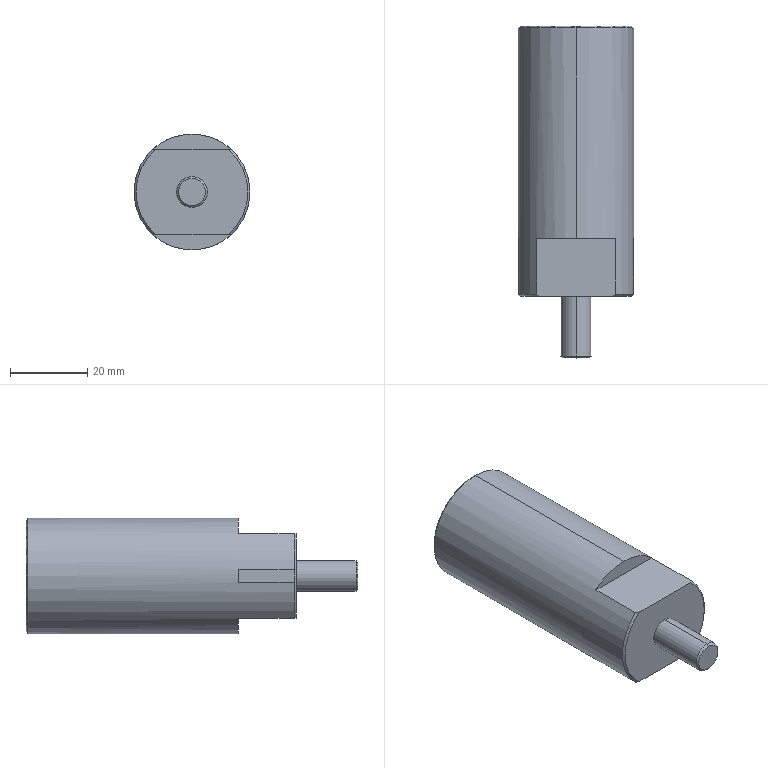Component | SolidWorks | MA060.03.03-11-10 | 1 solid | 25 faces | box 30 x 86 x 30 mm | volume 47690 mm3 | plane 11 | cone 8 | cylinder 6 | commonest cylinder face diameters 6.8 x2 8 x2 30 x2 | material Chrome Plated Round Bar
build123d program:
from build123d import *

# Parameters (mm, degrees)
M8_TAPPED_HOLE1_D     = 6.8
M8_TAPPED_HOLE1_DEPTH = 23.75
M8_TAPPED_HOLE1_TIP   = 2.043
CHAMFER1_SIZE         = 0.5
SKETCH4_OUTSIDE_W     = 51.18
SKETCH4_OUTSIDE_H     = 51.18
SKETCH4_OUTSIDE_W_2   = 22
SKETCH4_OUTSIDE_H_2   = 29.823
CUT_EXTRUDE1_DEPTH    = 15


with BuildPart() as part:
    # Sketch1 → Revolve1 (revolve)
    with BuildSketch(Plane.XY, mode=Mode.PRIVATE) as revolve1_sk:
        Polygon((0, 0), (0, 15), (70, 15), (70, 4), (86, 4), (86, 0), align=None)
    revolve(revolve1_sk.sketch.rotate(Axis((-16.338, 0, 0), (1, 0, 0)), 90), axis=Axis((-16.338, 0, 0), (1, 0, 0)))

    # M8 Tapped Hole1
    with Locations(Plane.ZY):
        with Locations((0, 0)):
            Hole(M8_TAPPED_HOLE1_D / 2, depth=M8_TAPPED_HOLE1_DEPTH)
            with Locations((0, 0, -(M8_TAPPED_HOLE1_DEPTH + M8_TAPPED_HOLE1_TIP / 2))):  # 118° drill point
                Cone(0, M8_TAPPED_HOLE1_D / 2, M8_TAPPED_HOLE1_TIP, mode=Mode.SUBTRACT)

    # Chamfer1
    chamfer1_edges = [part.edges().sort_by_distance(p)[0] for p in [
        (86, 0, -4),
        (70, 0, -15),
        (0, 0, -15),
    ]]
    chamfer(chamfer1_edges, length=CHAMFER1_SIZE)

    # Sketch4 outside → Cut-Extrude1 (cut)
    with BuildSketch(Plane(origin=(70, 0, 0), x_dir=(0, 0, -1), z_dir=(1, 0, 0))):
        Rectangle(SKETCH4_OUTSIDE_W, SKETCH4_OUTSIDE_H)
        Rectangle(SKETCH4_OUTSIDE_W_2, SKETCH4_OUTSIDE_H_2, mode=Mode.SUBTRACT)
    extrude(amount=-CUT_EXTRUDE1_DEPTH, mode=Mode.SUBTRACT)


solid = part.part

# Placed as in the assembly
solid = solid.moved(Location((-263.711, 172.053, 96.036), (0, 0, -90)))
STEP:
#1=COLOUR_RGB('',0.7922,0.8196,0.9333);
#2=FILL_AREA_STYLE_COLOUR('',#1);
#3=FILL_AREA_STYLE('',(#2));
#4=SURFACE_STYLE_FILL_AREA(#3);
#5=SURFACE_SIDE_STYLE('',(#4));
#6=SURFACE_STYLE_USAGE(.BOTH.,#5);
#7=PRESENTATION_STYLE_ASSIGNMENT((#6));
#8=CARTESIAN_POINT('',(-10.382,6.774,4.352));
#9=VERTEX_POINT('',#8);
#10=CARTESIAN_POINT('',(-10.382,6.774,3.21));
#11=VERTEX_POINT('',#10);
#12=CARTESIAN_POINT('',(-10.382,6.774,3.781));
#13=DIRECTION('',(-0.,1.,0.));
#14=DIRECTION('',(0.,0.,-1.));
#15=AXIS2_PLACEMENT_3D('',#12,#13,#14);
#16=CIRCLE('',#15,0.5709);
#17=EDGE_CURVE('',#9,#11,#16,.T.);
#18=ORIENTED_EDGE('',*,*,#17,.F.);
#19=CARTESIAN_POINT('',(-10.382,6.754,4.372));
#20=VERTEX_POINT('',#19);
#21=CARTESIAN_POINT('',(-10.382,6.774,4.352));
#22=DIRECTION('',(0.,-0.7071,0.7071));
#23=VECTOR('',#22,39.37);
#24=LINE('',#21,#23);
#25=EDGE_CURVE('',#9,#20,#24,.T.);
#26=ORIENTED_EDGE('',*,*,#25,.T.);
#27=CARTESIAN_POINT('',(-10.382,6.754,3.19));
#28=VERTEX_POINT('',#27);
#29=CARTESIAN_POINT('',(-10.382,6.754,3.781));
#30=DIRECTION('',(0.,-1.,-0.));
#31=DIRECTION('',(0.,0.,-1.));
#32=AXIS2_PLACEMENT_3D('',#29,#30,#31);
#33=CIRCLE('',#32,0.5906);
#34=EDGE_CURVE('',#28,#20,#33,.T.);
#35=ORIENTED_EDGE('',*,*,#34,.F.);
#36=CARTESIAN_POINT('',(-10.382,6.774,3.21));
#37=DIRECTION('',(0.,-0.7071,-0.7071));
#38=VECTOR('',#37,39.37);
#39=LINE('',#36,#38);
#40=EDGE_CURVE('',#11,#28,#39,.T.);
#41=ORIENTED_EDGE('',*,*,#40,.F.);
#42=EDGE_LOOP('',(#18,#26,#35,#41));
#43=FACE_OUTER_BOUND('',#42,.T.);
#44=CARTESIAN_POINT('',(-10.382,6.774,3.781));
#45=DIRECTION('',(0.,-1.,-0.));
#46=DIRECTION('',(0.,0.,-1.));
#47=AXIS2_PLACEMENT_3D('',#44,#45,#46);
#48=CONICAL_SURFACE('',#47,0.5709,0.7854);
#49=ADVANCED_FACE('',(#43),#48,.T.);
#50=CARTESIAN_POINT('',(-10.382,3.388,3.643));
#51=VERTEX_POINT('',#50);
#52=CARTESIAN_POINT('',(-10.382,3.388,3.919));
#53=VERTEX_POINT('',#52);
#54=CARTESIAN_POINT('',(-10.382,3.388,3.781));
#55=DIRECTION('',(0.,-1.,-0.));
#56=DIRECTION('',(0.,0.,1.));
#57=AXIS2_PLACEMENT_3D('',#54,#55,#56);
#58=CIRCLE('',#57,0.1378);
#59=EDGE_CURVE('',#51,#53,#58,.T.);
#60=ORIENTED_EDGE('',*,*,#59,.F.);
#61=CARTESIAN_POINT('',(-10.382,3.408,3.623));
#62=VERTEX_POINT('',#61);
#63=CARTESIAN_POINT('',(-10.382,3.408,3.623));
#64=DIRECTION('',(0.,0.7071,-0.7071));
#65=VECTOR('',#64,39.37);
#66=LINE('',#63,#65);
#67=EDGE_CURVE('',#51,#62,#66,.T.);
#68=ORIENTED_EDGE('',*,*,#67,.T.);
#69=CARTESIAN_POINT('',(-10.382,3.408,3.938));
#70=VERTEX_POINT('',#69);
#71=CARTESIAN_POINT('',(-10.382,3.408,3.781));
#72=DIRECTION('',(-0.,1.,0.));
#73=DIRECTION('',(0.,0.,1.));
#74=AXIS2_PLACEMENT_3D('',#71,#72,#73);
#75=CIRCLE('',#74,0.1575);
#76=EDGE_CURVE('',#70,#62,#75,.T.);
#77=ORIENTED_EDGE('',*,*,#76,.F.);
#78=CARTESIAN_POINT('',(-10.382,3.408,3.938));
#79=DIRECTION('',(-0.,0.7071,0.7071));
#80=VECTOR('',#79,39.37);
#81=LINE('',#78,#80);
#82=EDGE_CURVE('',#53,#70,#81,.T.);
#83=ORIENTED_EDGE('',*,*,#82,.F.);
#84=EDGE_LOOP('',(#60,#68,#77,#83));
#85=FACE_OUTER_BOUND('',#84,.T.);
#86=CARTESIAN_POINT('',(-10.382,3.408,3.781));
#87=DIRECTION('',(-0.,1.,0.));
#88=DIRECTION('',(0.,0.,1.));
#89=AXIS2_PLACEMENT_3D('',#86,#87,#88);
#90=CONICAL_SURFACE('',#89,0.1575,0.7854);
#91=ADVANCED_FACE('',(#85),#90,.T.);
#92=CARTESIAN_POINT('',(-10.382,5.839,3.647));
#93=VERTEX_POINT('',#92);
#94=CARTESIAN_POINT('',(-10.382,5.839,3.915));
#95=VERTEX_POINT('',#94);
#96=CARTESIAN_POINT('',(-10.382,5.839,3.781));
#97=DIRECTION('',(-0.,1.,0.));
#98=DIRECTION('',(0.,0.,1.));
#99=AXIS2_PLACEMENT_3D('',#96,#97,#98);
#100=CIRCLE('',#99,0.1339);
#101=EDGE_CURVE('',#93,#95,#100,.T.);
#102=ORIENTED_EDGE('',*,*,#101,.F.);
#103=CARTESIAN_POINT('',(-10.382,6.774,3.647));
#104=VERTEX_POINT('',#103);
#105=CARTESIAN_POINT('',(-10.382,6.774,3.647));
#106=DIRECTION('',(-0.,1.,0.));
#107=VECTOR('',#106,39.37);
#108=LINE('',#105,#107);
#109=EDGE_CURVE('',#93,#104,#108,.T.);
#110=ORIENTED_EDGE('',*,*,#109,.T.);
#111=CARTESIAN_POINT('',(-10.382,6.774,3.915));
#112=VERTEX_POINT('',#111);
#113=CARTESIAN_POINT('',(-10.382,6.774,3.781));
#114=DIRECTION('',(-0.,1.,0.));
#115=DIRECTION('',(0.,0.,1.));
#116=AXIS2_PLACEMENT_3D('',#113,#114,#115);
#117=CIRCLE('',#116,0.1339);
#118=EDGE_CURVE('',#104,#112,#117,.T.);
#119=ORIENTED_EDGE('',*,*,#118,.T.);
#120=CARTESIAN_POINT('',(-10.382,6.774,3.915));
#121=DIRECTION('',(-0.,1.,0.));
#122=VECTOR('',#121,39.37);
#123=LINE('',#120,#122);
#124=EDGE_CURVE('',#95,#112,#123,.T.);
#125=ORIENTED_EDGE('',*,*,#124,.F.);
#126=EDGE_LOOP('',(#102,#110,#119,#125));
#127=FACE_OUTER_BOUND('',#126,.T.);
#128=CARTESIAN_POINT('',(-10.382,6.774,3.781));
#129=DIRECTION('',(-0.,1.,0.));
#130=DIRECTION('',(0.,0.,1.));
#131=AXIS2_PLACEMENT_3D('',#128,#129,#130);
#132=CYLINDRICAL_SURFACE('',#131,0.1339);
#133=ADVANCED_FACE('',(#127),#132,.F.);
#134=CARTESIAN_POINT('',(-10.382,5.758,3.781));
#135=VERTEX_POINT('',#134);
#136=CARTESIAN_POINT('',(-10.382,5.839,3.915));
#137=DIRECTION('',(0.,0.515,0.8572));
#138=VECTOR('',#137,39.37);
#139=LINE('',#136,#138);
#140=EDGE_CURVE('',#135,#95,#139,.T.);
#141=ORIENTED_EDGE('',*,*,#140,.F.);
#142=CARTESIAN_POINT('',(-10.382,5.839,3.647));
#143=DIRECTION('',(0.,0.515,-0.8572));
#144=VECTOR('',#143,39.37);
#145=LINE('',#142,#144);
#146=EDGE_CURVE('',#135,#93,#145,.T.);
#147=ORIENTED_EDGE('',*,*,#146,.T.);
#148=ORIENTED_EDGE('',*,*,#101,.T.);
#149=EDGE_LOOP('',(#141,#147,#148));
#150=FACE_OUTER_BOUND('',#149,.T.);
#151=CARTESIAN_POINT('',(-10.382,5.839,3.781));
#152=DIRECTION('',(-0.,1.,0.));
#153=DIRECTION('',(0.,0.,1.));
#154=AXIS2_PLACEMENT_3D('',#151,#152,#153);
#155=CONICAL_SURFACE('',#154,0.1339,1.03);
#156=ADVANCED_FACE('',(#150),#155,.F.);
#157=ORIENTED_EDGE('',*,*,#76,.T.);
#158=CARTESIAN_POINT('',(-10.382,4.018,3.623));
#159=VERTEX_POINT('',#158);
#160=CARTESIAN_POINT('',(-10.382,7.417,3.623));
#161=DIRECTION('',(-0.,1.,0.));
#162=VECTOR('',#161,39.37);
#163=LINE('',#160,#162);
#164=EDGE_CURVE('',#62,#159,#163,.T.);
#165=ORIENTED_EDGE('',*,*,#164,.T.);
#166=CARTESIAN_POINT('',(-10.382,4.018,3.938));
#167=VERTEX_POINT('',#166);
#168=CARTESIAN_POINT('',(-10.382,4.018,3.781));
#169=DIRECTION('',(-0.,1.,0.));
#170=DIRECTION('',(0.,0.,1.));
#171=AXIS2_PLACEMENT_3D('',#168,#169,#170);
#172=CIRCLE('',#171,0.1575);
#173=EDGE_CURVE('',#167,#159,#172,.T.);
#174=ORIENTED_EDGE('',*,*,#173,.F.);
#175=CARTESIAN_POINT('',(-10.382,7.417,3.938));
#176=DIRECTION('',(-0.,1.,0.));
#177=VECTOR('',#176,39.37);
#178=LINE('',#175,#177);
#179=EDGE_CURVE('',#70,#167,#178,.T.);
#180=ORIENTED_EDGE('',*,*,#179,.F.);
#181=EDGE_LOOP('',(#157,#165,#174,#180));
#182=FACE_OUTER_BOUND('',#181,.T.);
#183=CARTESIAN_POINT('',(-10.382,7.417,3.781));
#184=DIRECTION('',(-0.,1.,0.));
#185=DIRECTION('',(0.,0.,1.));
#186=AXIS2_PLACEMENT_3D('',#183,#184,#185);
#187=CYLINDRICAL_SURFACE('',#186,0.1575);
#188=ADVANCED_FACE('',(#182),#187,.T.);
#189=CARTESIAN_POINT('',(-10.382,4.608,3.19));
#190=VERTEX_POINT('',#189);
#191=CARTESIAN_POINT('',(-9.981,4.608,3.348));
#192=VERTEX_POINT('',#191);
#193=CARTESIAN_POINT('',(-10.382,4.608,3.781));
#194=DIRECTION('',(0.,-1.,-0.));
#195=DIRECTION('',(0.,0.,-1.));
#196=AXIS2_PLACEMENT_3D('',#193,#194,#195);
#197=CIRCLE('',#196,0.5906);
#198=EDGE_CURVE('',#190,#192,#197,.T.);
#199=ORIENTED_EDGE('',*,*,#198,.F.);
#200=CARTESIAN_POINT('',(-10.382,7.417,3.19));
#201=DIRECTION('',(-0.,1.,0.));
#202=VECTOR('',#201,39.37);
#203=LINE('',#200,#202);
#204=EDGE_CURVE('',#190,#28,#203,.T.);
#205=ORIENTED_EDGE('',*,*,#204,.T.);
#206=ORIENTED_EDGE('',*,*,#34,.T.);
#207=CARTESIAN_POINT('',(-10.382,4.608,4.372));
#208=VERTEX_POINT('',#207);
#209=CARTESIAN_POINT('',(-10.382,7.417,4.372));
#210=DIRECTION('',(-0.,1.,0.));
#211=VECTOR('',#210,39.37);
#212=LINE('',#209,#211);
#213=EDGE_CURVE('',#208,#20,#212,.T.);
#214=ORIENTED_EDGE('',*,*,#213,.F.);
#215=CARTESIAN_POINT('',(-9.981,4.608,4.214));
#216=VERTEX_POINT('',#215);
#217=CARTESIAN_POINT('',(-10.382,4.608,3.781));
#218=DIRECTION('',(0.,-1.,-0.));
#219=DIRECTION('',(0.,0.,-1.));
#220=AXIS2_PLACEMENT_3D('',#217,#218,#219);
#221=CIRCLE('',#220,0.5906);
#222=EDGE_CURVE('',#216,#208,#221,.T.);
#223=ORIENTED_EDGE('',*,*,#222,.F.);
#224=CARTESIAN_POINT('',(-9.981,4.038,4.214));
#225=VERTEX_POINT('',#224);
#226=CARTESIAN_POINT('',(-9.981,7.417,4.214));
#227=DIRECTION('',(-0.,1.,0.));
#228=VECTOR('',#227,39.37);
#229=LINE('',#226,#228);
#230=EDGE_CURVE('',#225,#216,#229,.T.);
#231=ORIENTED_EDGE('',*,*,#230,.F.);
#232=CARTESIAN_POINT('',(-9.795,4.038,3.845));
#233=VERTEX_POINT('',#232);
#234=CARTESIAN_POINT('',(-10.382,4.038,3.781));
#235=DIRECTION('',(-0.,1.,0.));
#236=DIRECTION('',(0.,0.,1.));
#237=AXIS2_PLACEMENT_3D('',#234,#235,#236);
#238=CIRCLE('',#237,0.5906);
#239=EDGE_CURVE('',#225,#233,#238,.T.);
#240=ORIENTED_EDGE('',*,*,#239,.T.);
#241=CARTESIAN_POINT('',(-9.795,4.608,3.845));
#242=VERTEX_POINT('',#241);
#243=CARTESIAN_POINT('',(-9.795,7.417,3.845));
#244=DIRECTION('',(0.,-1.,-0.));
#245=VECTOR('',#244,39.37);
#246=LINE('',#243,#245);
#247=EDGE_CURVE('',#242,#233,#246,.T.);
#248=ORIENTED_EDGE('',*,*,#247,.F.);
#249=CARTESIAN_POINT('',(-9.795,4.608,3.717));
#250=VERTEX_POINT('',#249);
#251=CARTESIAN_POINT('',(-10.382,4.608,3.781));
#252=DIRECTION('',(0.,-1.,-0.));
#253=DIRECTION('',(0.,0.,-1.));
#254=AXIS2_PLACEMENT_3D('',#251,#252,#253);
#255=CIRCLE('',#254,0.5906);
#256=EDGE_CURVE('',#250,#242,#255,.T.);
#257=ORIENTED_EDGE('',*,*,#256,.F.);
#258=CARTESIAN_POINT('',(-9.795,4.038,3.717));
#259=VERTEX_POINT('',#258);
#260=CARTESIAN_POINT('',(-9.795,7.417,3.717));
#261=DIRECTION('',(-0.,1.,0.));
#262=VECTOR('',#261,39.37);
#263=LINE('',#260,#262);
#264=EDGE_CURVE('',#259,#250,#263,.T.);
#265=ORIENTED_EDGE('',*,*,#264,.F.);
#266=CARTESIAN_POINT('',(-9.981,4.038,3.348));
#267=VERTEX_POINT('',#266);
#268=CARTESIAN_POINT('',(-10.382,4.038,3.781));
#269=DIRECTION('',(-0.,1.,0.));
#270=DIRECTION('',(0.,0.,1.));
#271=AXIS2_PLACEMENT_3D('',#268,#269,#270);
#272=CIRCLE('',#271,0.5906);
#273=EDGE_CURVE('',#259,#267,#272,.T.);
#274=ORIENTED_EDGE('',*,*,#273,.T.);
#275=CARTESIAN_POINT('',(-9.981,7.417,3.348));
#276=DIRECTION('',(0.,-1.,-0.));
#277=VECTOR('',#276,39.37);
#278=LINE('',#275,#277);
#279=EDGE_CURVE('',#192,#267,#278,.T.);
#280=ORIENTED_EDGE('',*,*,#279,.F.);
#281=EDGE_LOOP('',(#199,#205,#206,#214,#223,#231,#240,#248,#257,#265,#274,#280));
#282=FACE_OUTER_BOUND('',#281,.T.);
#283=CARTESIAN_POINT('',(-10.382,7.417,3.781));
#284=DIRECTION('',(-0.,1.,0.));
#285=DIRECTION('',(0.,0.,1.));
#286=AXIS2_PLACEMENT_3D('',#283,#284,#285);
#287=CYLINDRICAL_SURFACE('',#286,0.5906);
#288=ADVANCED_FACE('',(#282),#287,.T.);
#289=ORIENTED_EDGE('',*,*,#204,.F.);
#290=CARTESIAN_POINT('',(-10.784,4.608,3.348));
#291=VERTEX_POINT('',#290);
#292=CARTESIAN_POINT('',(-10.382,4.608,3.781));
#293=DIRECTION('',(0.,-1.,-0.));
#294=DIRECTION('',(0.,0.,-1.));
#295=AXIS2_PLACEMENT_3D('',#292,#293,#294);
#296=CIRCLE('',#295,0.5906);
#297=EDGE_CURVE('',#291,#190,#296,.T.);
#298=ORIENTED_EDGE('',*,*,#297,.F.);
#299=CARTESIAN_POINT('',(-10.784,4.038,3.348));
#300=VERTEX_POINT('',#299);
#301=CARTESIAN_POINT('',(-10.784,7.417,3.348));
#302=DIRECTION('',(-0.,1.,0.));
#303=VECTOR('',#302,39.37);
#304=LINE('',#301,#303);
#305=EDGE_CURVE('',#300,#291,#304,.T.);
#306=ORIENTED_EDGE('',*,*,#305,.F.);
#307=CARTESIAN_POINT('',(-10.969,4.038,3.717));
#308=VERTEX_POINT('',#307);
#309=CARTESIAN_POINT('',(-10.382,4.038,3.781));
#310=DIRECTION('',(-0.,1.,0.));
#311=DIRECTION('',(0.,0.,1.));
#312=AXIS2_PLACEMENT_3D('',#309,#310,#311);
#313=CIRCLE('',#312,0.5906);
#314=EDGE_CURVE('',#300,#308,#313,.T.);
#315=ORIENTED_EDGE('',*,*,#314,.T.);
#316=CARTESIAN_POINT('',(-10.969,4.608,3.717));
#317=VERTEX_POINT('',#316);
#318=CARTESIAN_POINT('',(-10.969,7.417,3.717));
#319=DIRECTION('',(0.,-1.,-0.));
#320=VECTOR('',#319,39.37);
#321=LINE('',#318,#320);
#322=EDGE_CURVE('',#317,#308,#321,.T.);
#323=ORIENTED_EDGE('',*,*,#322,.F.);
#324=CARTESIAN_POINT('',(-10.969,4.608,3.845));
#325=VERTEX_POINT('',#324);
#326=CARTESIAN_POINT('',(-10.382,4.608,3.781));
#327=DIRECTION('',(0.,-1.,-0.));
#328=DIRECTION('',(0.,0.,-1.));
#329=AXIS2_PLACEMENT_3D('',#326,#327,#328);
#330=CIRCLE('',#329,0.5906);
#331=EDGE_CURVE('',#325,#317,#330,.T.);
#332=ORIENTED_EDGE('',*,*,#331,.F.);
#333=CARTESIAN_POINT('',(-10.969,4.038,3.845));
#334=VERTEX_POINT('',#333);
#335=CARTESIAN_POINT('',(-10.969,7.417,3.845));
#336=DIRECTION('',(-0.,1.,0.));
#337=VECTOR('',#336,39.37);
#338=LINE('',#335,#337);
#339=EDGE_CURVE('',#334,#325,#338,.T.);
#340=ORIENTED_EDGE('',*,*,#339,.F.);
#341=CARTESIAN_POINT('',(-10.784,4.038,4.214));
#342=VERTEX_POINT('',#341);
#343=CARTESIAN_POINT('',(-10.382,4.038,3.781));
#344=DIRECTION('',(-0.,1.,0.));
#345=DIRECTION('',(0.,0.,1.));
#346=AXIS2_PLACEMENT_3D('',#343,#344,#345);
#347=CIRCLE('',#346,0.5906);
#348=EDGE_CURVE('',#334,#342,#347,.T.);
#349=ORIENTED_EDGE('',*,*,#348,.T.);
#350=CARTESIAN_POINT('',(-10.784,4.608,4.214));
#351=VERTEX_POINT('',#350);
#352=CARTESIAN_POINT('',(-10.784,7.417,4.214));
#353=DIRECTION('',(0.,-1.,-0.));
#354=VECTOR('',#353,39.37);
#355=LINE('',#352,#354);
#356=EDGE_CURVE('',#351,#342,#355,.T.);
#357=ORIENTED_EDGE('',*,*,#356,.F.);
#358=CARTESIAN_POINT('',(-10.382,4.608,3.781));
#359=DIRECTION('',(0.,-1.,-0.));
#360=DIRECTION('',(0.,0.,-1.));
#361=AXIS2_PLACEMENT_3D('',#358,#359,#360);
#362=CIRCLE('',#361,0.5906);
#363=EDGE_CURVE('',#208,#351,#362,.T.);
#364=ORIENTED_EDGE('',*,*,#363,.F.);
#365=ORIENTED_EDGE('',*,*,#213,.T.);
#366=CARTESIAN_POINT('',(-10.382,6.754,3.781));
#367=DIRECTION('',(0.,-1.,-0.));
#368=DIRECTION('',(0.,0.,-1.));
#369=AXIS2_PLACEMENT_3D('',#366,#367,#368);
#370=CIRCLE('',#369,0.5906);
#371=EDGE_CURVE('',#20,#28,#370,.T.);
#372=ORIENTED_EDGE('',*,*,#371,.T.);
#373=EDGE_LOOP('',(#289,#298,#306,#315,#323,#332,#340,#349,#357,#364,#365,#372));
#374=FACE_OUTER_BOUND('',#373,.T.);
#375=CARTESIAN_POINT('',(-10.382,7.417,3.781));
#376=DIRECTION('',(-0.,1.,0.));
#377=DIRECTION('',(0.,0.,1.));
#378=AXIS2_PLACEMENT_3D('',#375,#376,#377);
#379=CYLINDRICAL_SURFACE('',#378,0.5906);
#380=ADVANCED_FACE('',(#374),#379,.T.);
#381=ORIENTED_EDGE('',*,*,#173,.T.);
#382=CARTESIAN_POINT('',(-10.382,4.018,3.781));
#383=DIRECTION('',(-0.,1.,0.));
#384=DIRECTION('',(0.,0.,1.));
#385=AXIS2_PLACEMENT_3D('',#382,#383,#384);
#386=CIRCLE('',#385,0.1575);
#387=EDGE_CURVE('',#159,#167,#386,.T.);
#388=ORIENTED_EDGE('',*,*,#387,.T.);
#389=EDGE_LOOP('',(#381,#388));
#390=FACE_BOUND('',#389,.T.);
#391=CARTESIAN_POINT('',(-10.754,4.018,3.348));
#392=VERTEX_POINT('',#391);
#393=CARTESIAN_POINT('',(-10.01,4.018,3.348));
#394=VERTEX_POINT('',#393);
#395=CARTESIAN_POINT('',(-10.969,4.018,3.348));
#396=DIRECTION('',(1.,0.,-0.));
#397=VECTOR('',#396,39.37);
#398=LINE('',#395,#397);
#399=EDGE_CURVE('',#392,#394,#398,.T.);
#400=ORIENTED_EDGE('',*,*,#399,.T.);
#401=CARTESIAN_POINT('',(-10.01,4.018,4.214));
#402=VERTEX_POINT('',#401);
#403=CARTESIAN_POINT('',(-10.382,4.018,3.781));
#404=DIRECTION('',(0.,-1.,-0.));
#405=DIRECTION('',(0.,0.,1.));
#406=AXIS2_PLACEMENT_3D('',#403,#404,#405);
#407=CIRCLE('',#406,0.5709);
#408=EDGE_CURVE('',#394,#402,#407,.T.);
#409=ORIENTED_EDGE('',*,*,#408,.T.);
#410=CARTESIAN_POINT('',(-10.754,4.018,4.214));
#411=VERTEX_POINT('',#410);
#412=CARTESIAN_POINT('',(-10.969,4.018,4.214));
#413=DIRECTION('',(-1.,-0.,0.));
#414=VECTOR('',#413,39.37);
#415=LINE('',#412,#414);
#416=EDGE_CURVE('',#402,#411,#415,.T.);
#417=ORIENTED_EDGE('',*,*,#416,.T.);
#418=CARTESIAN_POINT('',(-10.382,4.018,3.781));
#419=DIRECTION('',(0.,-1.,-0.));
#420=DIRECTION('',(0.,0.,1.));
#421=AXIS2_PLACEMENT_3D('',#418,#419,#420);
#422=CIRCLE('',#421,0.5709);
#423=EDGE_CURVE('',#411,#392,#422,.T.);
#424=ORIENTED_EDGE('',*,*,#423,.T.);
#425=EDGE_LOOP('',(#400,#409,#417,#424));
#426=FACE_OUTER_BOUND('',#425,.T.);
#427=CARTESIAN_POINT('',(-9.792,4.018,3.781));
#428=DIRECTION('',(-0.,1.,0.));
#429=DIRECTION('',(0.,-0.,1.));
#430=AXIS2_PLACEMENT_3D('',#427,#428,#429);
#431=PLANE('',#430);
#432=ADVANCED_FACE('',(#390,#426),#431,.F.);
#433=ORIENTED_EDGE('',*,*,#314,.F.);
#434=CARTESIAN_POINT('',(-10.784,4.038,3.348));
#435=CARTESIAN_POINT('',(-10.774,4.031,3.348));
#436=CARTESIAN_POINT('',(-10.764,4.024,3.348));
#437=CARTESIAN_POINT('',(-10.754,4.018,3.348));
#438=B_SPLINE_CURVE_WITH_KNOTS('',3,(#434,#435,#436,#437),.UNSPECIFIED.,.F.,.F.,(4,4),(0.02749,0.0284),.UNSPECIFIED.);
#439=EDGE_CURVE('',#300,#392,#438,.T.);
#440=ORIENTED_EDGE('',*,*,#439,.T.);
#441=ORIENTED_EDGE('',*,*,#423,.F.);
#442=CARTESIAN_POINT('',(-10.754,4.018,4.214));
#443=CARTESIAN_POINT('',(-10.764,4.024,4.214));
#444=CARTESIAN_POINT('',(-10.774,4.031,4.214));
#445=CARTESIAN_POINT('',(-10.784,4.038,4.214));
#446=B_SPLINE_CURVE_WITH_KNOTS('',3,(#442,#443,#444,#445),.UNSPECIFIED.,.F.,.F.,(4,4),(0.04866,0.04955),.UNSPECIFIED.);
#447=EDGE_CURVE('',#411,#342,#446,.T.);
#448=ORIENTED_EDGE('',*,*,#447,.T.);
#449=ORIENTED_EDGE('',*,*,#348,.F.);
#450=CARTESIAN_POINT('',(-10.969,4.038,3.845));
#451=CARTESIAN_POINT('',(-10.969,4.033,3.802));
#452=CARTESIAN_POINT('',(-10.969,4.033,3.759));
#453=CARTESIAN_POINT('',(-10.969,4.038,3.717));
#454=B_SPLINE_CURVE_WITH_KNOTS('',3,(#450,#451,#452,#453),.UNSPECIFIED.,.F.,.F.,(4,4),(0.006529,0.009767),.UNSPECIFIED.);
#455=EDGE_CURVE('',#334,#308,#454,.T.);
#456=ORIENTED_EDGE('',*,*,#455,.T.);
#457=EDGE_LOOP('',(#433,#440,#441,#448,#449,#456));
#458=FACE_OUTER_BOUND('',#457,.T.);
#459=CARTESIAN_POINT('',(-10.382,4.038,3.781));
#460=DIRECTION('',(-0.,1.,0.));
#461=DIRECTION('',(0.,0.,1.));
#462=AXIS2_PLACEMENT_3D('',#459,#460,#461);
#463=CONICAL_SURFACE('',#462,0.5906,0.7854);
#464=ADVANCED_FACE('',(#458),#463,.T.);
#465=ORIENTED_EDGE('',*,*,#408,.F.);
#466=CARTESIAN_POINT('',(-10.01,4.018,3.348));
#467=CARTESIAN_POINT('',(-10.,4.024,3.348));
#468=CARTESIAN_POINT('',(-9.991,4.031,3.348));
#469=CARTESIAN_POINT('',(-9.981,4.038,3.348));
#470=B_SPLINE_CURVE_WITH_KNOTS('',3,(#466,#467,#468,#469),.UNSPECIFIED.,.F.,.F.,(4,4),(0.04866,0.04955),.UNSPECIFIED.);
#471=EDGE_CURVE('',#394,#267,#470,.T.);
#472=ORIENTED_EDGE('',*,*,#471,.T.);
#473=ORIENTED_EDGE('',*,*,#273,.F.);
#474=CARTESIAN_POINT('',(-9.795,4.038,3.717));
#475=CARTESIAN_POINT('',(-9.795,4.033,3.759));
#476=CARTESIAN_POINT('',(-9.795,4.033,3.802));
#477=CARTESIAN_POINT('',(-9.795,4.038,3.845));
#478=B_SPLINE_CURVE_WITH_KNOTS('',3,(#474,#475,#476,#477),.UNSPECIFIED.,.F.,.F.,(4,4),(0.007731,0.01097),.UNSPECIFIED.);
#479=EDGE_CURVE('',#259,#233,#478,.T.);
#480=ORIENTED_EDGE('',*,*,#479,.T.);
#481=ORIENTED_EDGE('',*,*,#239,.F.);
#482=CARTESIAN_POINT('',(-9.981,4.038,4.214));
#483=CARTESIAN_POINT('',(-9.991,4.031,4.214));
#484=CARTESIAN_POINT('',(-10.,4.024,4.214));
#485=CARTESIAN_POINT('',(-10.01,4.018,4.214));
#486=B_SPLINE_CURVE_WITH_KNOTS('',3,(#482,#483,#484,#485),.UNSPECIFIED.,.F.,.F.,(4,4),(0.02749,0.0284),.UNSPECIFIED.);
#487=EDGE_CURVE('',#225,#402,#486,.T.);
#488=ORIENTED_EDGE('',*,*,#487,.T.);
#489=EDGE_LOOP('',(#465,#472,#473,#480,#481,#488));
#490=FACE_OUTER_BOUND('',#489,.T.);
#491=CARTESIAN_POINT('',(-10.382,4.038,3.781));
#492=DIRECTION('',(-0.,1.,0.));
#493=DIRECTION('',(0.,0.,1.));
#494=AXIS2_PLACEMENT_3D('',#491,#492,#493);
#495=CONICAL_SURFACE('',#494,0.5906,0.7854);
#496=ADVANCED_FACE('',(#490),#495,.T.);
#497=CARTESIAN_POINT('',(-10.382,6.774,3.781));
#498=DIRECTION('',(-0.,1.,0.));
#499=DIRECTION('',(0.,0.,-1.));
#500=AXIS2_PLACEMENT_3D('',#497,#498,#499);
#501=CIRCLE('',#500,0.5709);
#502=EDGE_CURVE('',#11,#9,#501,.T.);
#503=ORIENTED_EDGE('',*,*,#502,.T.);
#504=ORIENTED_EDGE('',*,*,#17,.T.);
#505=EDGE_LOOP('',(#503,#504));
#506=FACE_OUTER_BOUND('',#505,.T.);
#507=CARTESIAN_POINT('',(-10.382,6.774,3.781));
#508=DIRECTION('',(-0.,1.,0.));
#509=DIRECTION('',(0.,0.,1.));
#510=AXIS2_PLACEMENT_3D('',#507,#508,#509);
#511=CIRCLE('',#510,0.1339);
#512=EDGE_CURVE('',#112,#104,#511,.T.);
#513=ORIENTED_EDGE('',*,*,#512,.F.);
#514=ORIENTED_EDGE('',*,*,#118,.F.);
#515=EDGE_LOOP('',(#513,#514));
#516=FACE_BOUND('',#515,.T.);
#517=CARTESIAN_POINT('',(-10.382,6.774,3.781));
#518=DIRECTION('',(0.,-1.,-0.));
#519=DIRECTION('',(-0.,0.,-1.));
#520=AXIS2_PLACEMENT_3D('',#517,#518,#519);
#521=PLANE('',#520);
#522=ADVANCED_FACE('',(#506,#516),#521,.F.);
#523=ORIENTED_EDGE('',*,*,#164,.F.);
#524=CARTESIAN_POINT('',(-10.382,3.408,3.781));
#525=DIRECTION('',(-0.,1.,0.));
#526=DIRECTION('',(0.,0.,1.));
#527=AXIS2_PLACEMENT_3D('',#524,#525,#526);
#528=CIRCLE('',#527,0.1575);
#529=EDGE_CURVE('',#62,#70,#528,.T.);
#530=ORIENTED_EDGE('',*,*,#529,.T.);
#531=ORIENTED_EDGE('',*,*,#179,.T.);
#532=ORIENTED_EDGE('',*,*,#387,.F.);
#533=EDGE_LOOP('',(#523,#530,#531,#532));
#534=FACE_OUTER_BOUND('',#533,.T.);
#535=CARTESIAN_POINT('',(-10.382,7.417,3.781));
#536=DIRECTION('',(-0.,1.,0.));
#537=DIRECTION('',(0.,0.,1.));
#538=AXIS2_PLACEMENT_3D('',#535,#536,#537);
#539=CYLINDRICAL_SURFACE('',#538,0.1575);
#540=ADVANCED_FACE('',(#534),#539,.T.);
#541=CARTESIAN_POINT('',(-10.382,3.388,3.781));
#542=DIRECTION('',(0.,-1.,-0.));
#543=DIRECTION('',(0.,0.,1.));
#544=AXIS2_PLACEMENT_3D('',#541,#542,#543);
#545=CIRCLE('',#544,0.1378);
#546=EDGE_CURVE('',#53,#51,#545,.T.);
#547=ORIENTED_EDGE('',*,*,#546,.T.);
#548=ORIENTED_EDGE('',*,*,#59,.T.);
#549=EDGE_LOOP('',(#547,#548));
#550=FACE_OUTER_BOUND('',#549,.T.);
#551=CARTESIAN_POINT('',(-10.225,3.388,3.781));
#552=DIRECTION('',(-0.,1.,0.));
#553=DIRECTION('',(0.,-0.,1.));
#554=AXIS2_PLACEMENT_3D('',#551,#552,#553);
#555=PLANE('',#554);
#556=ADVANCED_FACE('',(#550),#555,.F.);
#557=ORIENTED_EDGE('',*,*,#146,.F.);
#558=ORIENTED_EDGE('',*,*,#140,.T.);
#559=CARTESIAN_POINT('',(-10.382,5.839,3.781));
#560=DIRECTION('',(-0.,1.,0.));
#561=DIRECTION('',(0.,0.,1.));
#562=AXIS2_PLACEMENT_3D('',#559,#560,#561);
#563=CIRCLE('',#562,0.1339);
#564=EDGE_CURVE('',#95,#93,#563,.T.);
#565=ORIENTED_EDGE('',*,*,#564,.T.);
#566=EDGE_LOOP('',(#557,#558,#565));
#567=FACE_OUTER_BOUND('',#566,.T.);
#568=CARTESIAN_POINT('',(-10.382,5.839,3.781));
#569=DIRECTION('',(-0.,1.,0.));
#570=DIRECTION('',(0.,0.,1.));
#571=AXIS2_PLACEMENT_3D('',#568,#569,#570);
#572=CONICAL_SURFACE('',#571,0.1339,1.03);
#573=ADVANCED_FACE('',(#567),#572,.F.);
#574=ORIENTED_EDGE('',*,*,#109,.F.);
#575=ORIENTED_EDGE('',*,*,#564,.F.);
#576=ORIENTED_EDGE('',*,*,#124,.T.);
#577=ORIENTED_EDGE('',*,*,#512,.T.);
#578=EDGE_LOOP('',(#574,#575,#576,#577));
#579=FACE_OUTER_BOUND('',#578,.T.);
#580=CARTESIAN_POINT('',(-10.382,6.774,3.781));
#581=DIRECTION('',(-0.,1.,0.));
#582=DIRECTION('',(0.,0.,1.));
#583=AXIS2_PLACEMENT_3D('',#580,#581,#582);
#584=CYLINDRICAL_SURFACE('',#583,0.1339);
#585=ADVANCED_FACE('',(#579),#584,.F.);
#586=ORIENTED_EDGE('',*,*,#67,.F.);
#587=ORIENTED_EDGE('',*,*,#546,.F.);
#588=ORIENTED_EDGE('',*,*,#82,.T.);
#589=ORIENTED_EDGE('',*,*,#529,.F.);
#590=EDGE_LOOP('',(#586,#587,#588,#589));
#591=FACE_OUTER_BOUND('',#590,.T.);
#592=CARTESIAN_POINT('',(-10.382,3.408,3.781));
#593=DIRECTION('',(-0.,1.,0.));
#594=DIRECTION('',(0.,0.,1.));
#595=AXIS2_PLACEMENT_3D('',#592,#593,#594);
#596=CONICAL_SURFACE('',#595,0.1575,0.7854);
#597=ADVANCED_FACE('',(#591),#596,.T.);
#598=ORIENTED_EDGE('',*,*,#25,.F.);
#599=ORIENTED_EDGE('',*,*,#502,.F.);
#600=ORIENTED_EDGE('',*,*,#40,.T.);
#601=ORIENTED_EDGE('',*,*,#371,.F.);
#602=EDGE_LOOP('',(#598,#599,#600,#601));
#603=FACE_OUTER_BOUND('',#602,.T.);
#604=CARTESIAN_POINT('',(-10.382,6.774,3.781));
#605=DIRECTION('',(0.,-1.,-0.));
#606=DIRECTION('',(0.,0.,-1.));
#607=AXIS2_PLACEMENT_3D('',#604,#605,#606);
#608=CONICAL_SURFACE('',#607,0.5709,0.7854);
#609=ADVANCED_FACE('',(#603),#608,.T.);
#610=ORIENTED_EDGE('',*,*,#264,.T.);
#611=CARTESIAN_POINT('',(-9.795,4.608,4.214));
#612=DIRECTION('',(0.,-0.,1.));
#613=VECTOR('',#612,39.37);
#614=LINE('',#611,#613);
#615=EDGE_CURVE('',#250,#242,#614,.T.);
#616=ORIENTED_EDGE('',*,*,#615,.T.);
#617=ORIENTED_EDGE('',*,*,#247,.T.);
#618=ORIENTED_EDGE('',*,*,#479,.F.);
#619=EDGE_LOOP('',(#610,#616,#617,#618));
#620=FACE_OUTER_BOUND('',#619,.T.);
#621=CARTESIAN_POINT('',(-9.795,4.608,4.214));
#622=DIRECTION('',(1.,0.,-0.));
#623=DIRECTION('',(0.,-0.,1.));
#624=AXIS2_PLACEMENT_3D('',#621,#622,#623);
#625=PLANE('',#624);
#626=ADVANCED_FACE('',(#620),#625,.T.);
#627=ORIENTED_EDGE('',*,*,#256,.T.);
#628=ORIENTED_EDGE('',*,*,#615,.F.);
#629=EDGE_LOOP('',(#627,#628));
#630=FACE_OUTER_BOUND('',#629,.T.);
#631=CARTESIAN_POINT('',(-10.382,4.608,3.781));
#632=DIRECTION('',(0.,-1.,-0.));
#633=DIRECTION('',(-0.,0.,-1.));
#634=AXIS2_PLACEMENT_3D('',#631,#632,#633);
#635=PLANE('',#634);
#636=ADVANCED_FACE('',(#630),#635,.T.);
#637=ORIENTED_EDGE('',*,*,#230,.T.);
#638=CARTESIAN_POINT('',(-10.969,4.608,4.214));
#639=DIRECTION('',(-1.,-0.,0.));
#640=VECTOR('',#639,39.37);
#641=LINE('',#638,#640);
#642=EDGE_CURVE('',#216,#351,#641,.T.);
#643=ORIENTED_EDGE('',*,*,#642,.T.);
#644=ORIENTED_EDGE('',*,*,#356,.T.);
#645=ORIENTED_EDGE('',*,*,#447,.F.);
#646=ORIENTED_EDGE('',*,*,#416,.F.);
#647=ORIENTED_EDGE('',*,*,#487,.F.);
#648=EDGE_LOOP('',(#637,#643,#644,#645,#646,#647));
#649=FACE_OUTER_BOUND('',#648,.T.);
#650=CARTESIAN_POINT('',(-10.969,4.608,4.214));
#651=DIRECTION('',(0.,-0.,1.));
#652=DIRECTION('',(0.,-1.,-0.));
#653=AXIS2_PLACEMENT_3D('',#650,#651,#652);
#654=PLANE('',#653);
#655=ADVANCED_FACE('',(#649),#654,.T.);
#656=ORIENTED_EDGE('',*,*,#222,.T.);
#657=ORIENTED_EDGE('',*,*,#363,.T.);
#658=ORIENTED_EDGE('',*,*,#642,.F.);
#659=EDGE_LOOP('',(#656,#657,#658));
#660=FACE_OUTER_BOUND('',#659,.T.);
#661=CARTESIAN_POINT('',(-10.382,4.608,3.781));
#662=DIRECTION('',(0.,-1.,-0.));
#663=DIRECTION('',(-0.,0.,-1.));
#664=AXIS2_PLACEMENT_3D('',#661,#662,#663);
#665=PLANE('',#664);
#666=ADVANCED_FACE('',(#660),#665,.T.);
#667=ORIENTED_EDGE('',*,*,#339,.T.);
#668=CARTESIAN_POINT('',(-10.969,4.608,4.214));
#669=DIRECTION('',(-0.,0.,-1.));
#670=VECTOR('',#669,39.37);
#671=LINE('',#668,#670);
#672=EDGE_CURVE('',#325,#317,#671,.T.);
#673=ORIENTED_EDGE('',*,*,#672,.T.);
#674=ORIENTED_EDGE('',*,*,#322,.T.);
#675=ORIENTED_EDGE('',*,*,#455,.F.);
#676=EDGE_LOOP('',(#667,#673,#674,#675));
#677=FACE_OUTER_BOUND('',#676,.T.);
#678=CARTESIAN_POINT('',(-10.969,4.608,4.214));
#679=DIRECTION('',(-1.,-0.,0.));
#680=DIRECTION('',(-0.,0.,-1.));
#681=AXIS2_PLACEMENT_3D('',#678,#679,#680);
#682=PLANE('',#681);
#683=ADVANCED_FACE('',(#677),#682,.T.);
#684=ORIENTED_EDGE('',*,*,#331,.T.);
#685=ORIENTED_EDGE('',*,*,#672,.F.);
#686=EDGE_LOOP('',(#684,#685));
#687=FACE_OUTER_BOUND('',#686,.T.);
#688=CARTESIAN_POINT('',(-10.382,4.608,3.781));
#689=DIRECTION('',(0.,-1.,-0.));
#690=DIRECTION('',(-0.,0.,-1.));
#691=AXIS2_PLACEMENT_3D('',#688,#689,#690);
#692=PLANE('',#691);
#693=ADVANCED_FACE('',(#687),#692,.T.);
#694=ORIENTED_EDGE('',*,*,#297,.T.);
#695=ORIENTED_EDGE('',*,*,#198,.T.);
#696=CARTESIAN_POINT('',(-10.969,4.608,3.348));
#697=DIRECTION('',(1.,0.,-0.));
#698=VECTOR('',#697,39.37);
#699=LINE('',#696,#698);
#700=EDGE_CURVE('',#291,#192,#699,.T.);
#701=ORIENTED_EDGE('',*,*,#700,.F.);
#702=EDGE_LOOP('',(#694,#695,#701));
#703=FACE_OUTER_BOUND('',#702,.T.);
#704=CARTESIAN_POINT('',(-10.382,4.608,3.781));
#705=DIRECTION('',(0.,-1.,-0.));
#706=DIRECTION('',(-0.,0.,-1.));
#707=AXIS2_PLACEMENT_3D('',#704,#705,#706);
#708=PLANE('',#707);
#709=ADVANCED_FACE('',(#703),#708,.T.);
#710=ORIENTED_EDGE('',*,*,#305,.T.);
#711=ORIENTED_EDGE('',*,*,#700,.T.);
#712=ORIENTED_EDGE('',*,*,#279,.T.);
#713=ORIENTED_EDGE('',*,*,#471,.F.);
#714=ORIENTED_EDGE('',*,*,#399,.F.);
#715=ORIENTED_EDGE('',*,*,#439,.F.);
#716=EDGE_LOOP('',(#710,#711,#712,#713,#714,#715));
#717=FACE_OUTER_BOUND('',#716,.T.);
#718=CARTESIAN_POINT('',(-10.969,4.608,3.348));
#719=DIRECTION('',(-0.,0.,-1.));
#720=DIRECTION('',(-0.,1.,0.));
#721=AXIS2_PLACEMENT_3D('',#718,#719,#720);
#722=PLANE('',#721);
#723=ADVANCED_FACE('',(#717),#722,.T.);
#724=CLOSED_SHELL('',(#49,#91,#133,#156,#188,#288,#380,#432,#464,#496,#522,#540,#556,#573,#585,#597,#609,#626,#636,#655,#666,#683,#693,#709,#723));
#725=MANIFOLD_SOLID_BREP('',#724);
#726=STYLED_ITEM('',(#7),#725);
#727=PRESENTATION_LAYER_ASSIGNMENT('','',(#726));
#728=(LENGTH_UNIT()NAMED_UNIT(*)SI_UNIT($,.METRE.));
#729=LENGTH_MEASURE_WITH_UNIT(LENGTH_MEASURE(0.0254),#728);
#730=DIMENSIONAL_EXPONENTS(1.,0.,0.,0.,0.,0.,0.);
#731=(CONVERSION_BASED_UNIT('',#729)LENGTH_UNIT()NAMED_UNIT(#730));
#732=UNCERTAINTY_MEASURE_WITH_UNIT(LENGTH_MEASURE(0.00001),#731,'','');
#733=(NAMED_UNIT(*)PLANE_ANGLE_UNIT()SI_UNIT($,.RADIAN.));
#734=(NAMED_UNIT(*)SI_UNIT($,.STERADIAN.)SOLID_ANGLE_UNIT());
#735=(GEOMETRIC_REPRESENTATION_CONTEXT(3)GLOBAL_UNCERTAINTY_ASSIGNED_CONTEXT((#732))GLOBAL_UNIT_ASSIGNED_CONTEXT((#731,#733,#734))REPRESENTATION_CONTEXT('',''));
#736=MECHANICAL_DESIGN_GEOMETRIC_PRESENTATION_REPRESENTATION('',(#726),#735);
#737=CARTESIAN_POINT('',(0.,0.,0.));
#738=DIRECTION('',(0.,0.,1.));
#739=DIRECTION('',(1.,0.,0.));
#740=AXIS2_PLACEMENT_3D('',#737,#738,#739);
#741=(LENGTH_UNIT()NAMED_UNIT(*)SI_UNIT($,.METRE.));
#742=LENGTH_MEASURE_WITH_UNIT(LENGTH_MEASURE(0.0254),#741);
#743=DIMENSIONAL_EXPONENTS(1.,0.,0.,0.,0.,0.,0.);
#744=(CONVERSION_BASED_UNIT('',#742)LENGTH_UNIT()NAMED_UNIT(#743));
#745=UNCERTAINTY_MEASURE_WITH_UNIT(LENGTH_MEASURE(0.00001),#744,'','');
#746=(NAMED_UNIT(*)PLANE_ANGLE_UNIT()SI_UNIT($,.RADIAN.));
#747=(NAMED_UNIT(*)SI_UNIT($,.STERADIAN.)SOLID_ANGLE_UNIT());
#748=(GEOMETRIC_REPRESENTATION_CONTEXT(3)GLOBAL_UNCERTAINTY_ASSIGNED_CONTEXT((#745))GLOBAL_UNIT_ASSIGNED_CONTEXT((#744,#746,#747))REPRESENTATION_CONTEXT('',''));
#749=ADVANCED_BREP_SHAPE_REPRESENTATION('',(#725,#740),#748);